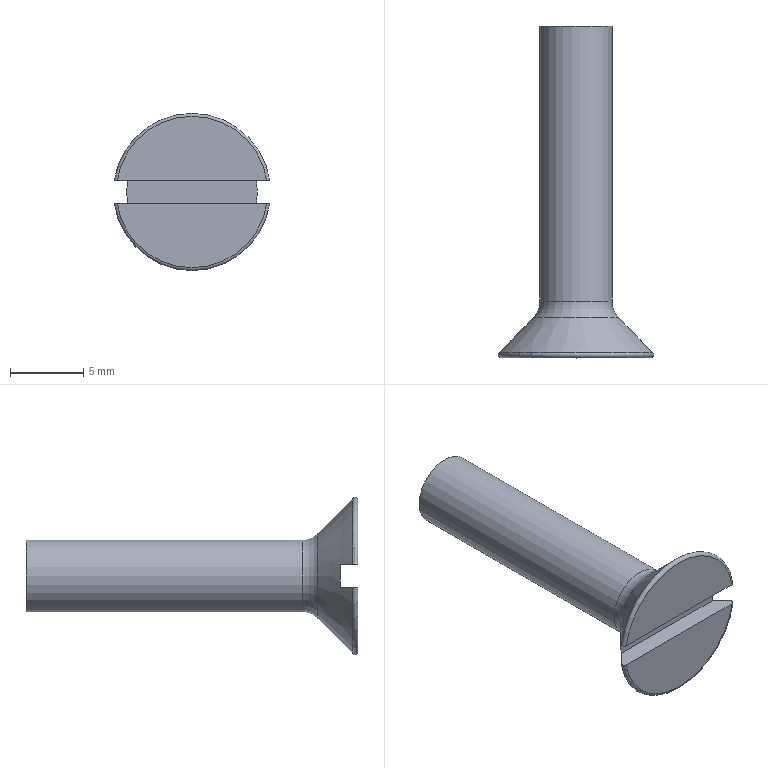Component | NX | SCREW_M6X18 | 1 solid | 11 faces | volume 523 mm3 | plane 6 | torus 3 | cylinder 1 | cone 1 | commonest cylinder face diameters 4.917 x1